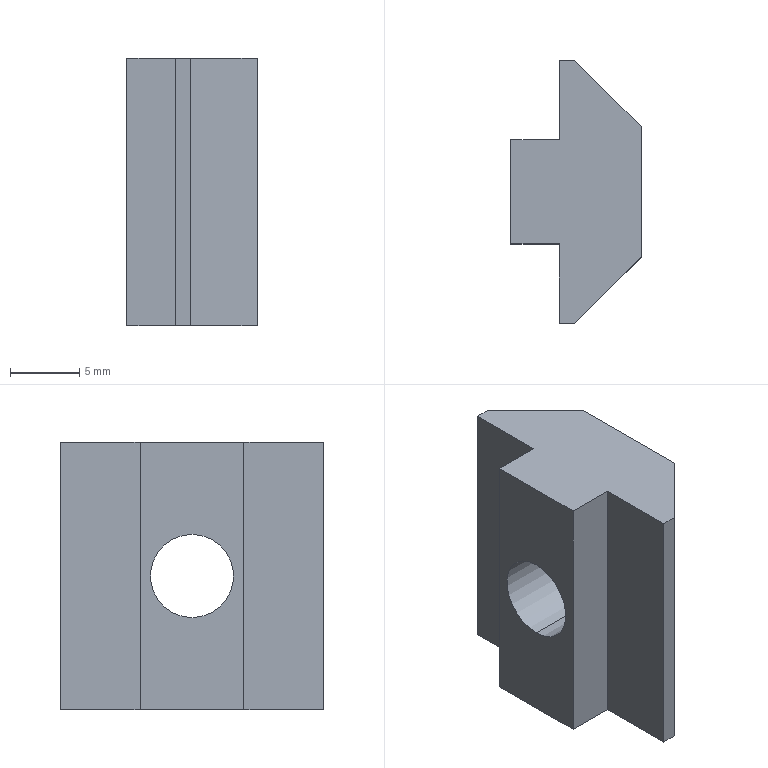Component | SolidWorks | SquareNutBlock-MC6-8-30-1 | 1 solid | 14 faces | box 9.4 x 19 x 19.3 mm | volume 1960 mm3 | plane 12 | cylinder 2 | commonest cylinder face diameters 6 x2 | material Purchased Part
build123d program:
from build123d import *

# Parameters (mm, degrees)
BOSS_EXTRUDE1_DEPTH = 9.65
M6_TAPPED_HOLE1_D   = 6


with BuildPart() as part:
    # Sketch1 → Boss-Extrude1 (new, symmetric)
    with BuildSketch(Plane.XY):
        Polygon((0, -3.75), (0, 3.75), (3.5, 3.75), (3.5, 9.5), (4.6, 9.5), (9.4, 4.7), (9.4, -4.7), (4.6, -9.5), (3.5, -9.5), (3.5, -3.75), align=None)
    extrude(amount=BOSS_EXTRUDE1_DEPTH, both=True)

    # M6 Tapped Hole1 (through all)
    with Locations(Plane(origin=(9.4, 0, 0), x_dir=(0, 0, -1), z_dir=(1, 0, 0))):
        with Locations((0, 0)):
            Hole(M6_TAPPED_HOLE1_D / 2)


solid = part.part

# Placed as in the assembly
solid = solid.moved(Location((11.4, -250, 10), (0, 0, 0)))
STEP:
#1=CARTESIAN_POINT('',(0.4488,-9.843,0.5118));
#2=VERTEX_POINT('',#1);
#3=CARTESIAN_POINT('',(0.4488,-9.843,0.2756));
#4=VERTEX_POINT('',#3);
#5=CARTESIAN_POINT('',(0.4488,-9.843,0.3937));
#6=DIRECTION('',(1.,0.,0.));
#7=DIRECTION('',(0.,0.,-1.));
#8=AXIS2_PLACEMENT_3D('',#5,#6,#7);
#9=CIRCLE('',#8,0.1181);
#10=EDGE_CURVE('',#2,#4,#9,.T.);
#11=ORIENTED_EDGE('',*,*,#10,.F.);
#12=CARTESIAN_POINT('',(0.8189,-9.843,0.5118));
#13=VERTEX_POINT('',#12);
#14=CARTESIAN_POINT('',(0.8189,-9.843,0.5118));
#15=DIRECTION('',(1.,0.,0.));
#16=VECTOR('',#15,39.37);
#17=LINE('',#14,#16);
#18=EDGE_CURVE('',#2,#13,#17,.T.);
#19=ORIENTED_EDGE('',*,*,#18,.T.);
#20=CARTESIAN_POINT('',(0.8189,-9.843,0.2756));
#21=VERTEX_POINT('',#20);
#22=CARTESIAN_POINT('',(0.8189,-9.843,0.3937));
#23=DIRECTION('',(1.,0.,0.));
#24=DIRECTION('',(0.,0.,-1.));
#25=AXIS2_PLACEMENT_3D('',#22,#23,#24);
#26=CIRCLE('',#25,0.1181);
#27=EDGE_CURVE('',#13,#21,#26,.T.);
#28=ORIENTED_EDGE('',*,*,#27,.T.);
#29=CARTESIAN_POINT('',(0.8189,-9.843,0.2756));
#30=DIRECTION('',(1.,0.,0.));
#31=VECTOR('',#30,39.37);
#32=LINE('',#29,#31);
#33=EDGE_CURVE('',#4,#21,#32,.T.);
#34=ORIENTED_EDGE('',*,*,#33,.F.);
#35=EDGE_LOOP('',(#11,#19,#28,#34));
#36=FACE_OUTER_BOUND('',#35,.T.);
#37=CARTESIAN_POINT('',(0.8189,-9.843,0.3937));
#38=DIRECTION('',(1.,0.,0.));
#39=DIRECTION('',(0.,0.,-1.));
#40=AXIS2_PLACEMENT_3D('',#37,#38,#39);
#41=CYLINDRICAL_SURFACE('',#40,0.1181);
#42=ADVANCED_FACE('',(#36),#41,.F.);
#43=CARTESIAN_POINT('',(0.4488,-9.99,0.01378));
#44=VERTEX_POINT('',#43);
#45=CARTESIAN_POINT('',(0.5866,-9.99,0.01378));
#46=VERTEX_POINT('',#45);
#47=CARTESIAN_POINT('',(0.5866,-9.99,0.01378));
#48=DIRECTION('',(1.,0.,0.));
#49=VECTOR('',#48,39.37);
#50=LINE('',#47,#49);
#51=EDGE_CURVE('',#44,#46,#50,.T.);
#52=ORIENTED_EDGE('',*,*,#51,.T.);
#53=CARTESIAN_POINT('',(0.5866,-9.99,0.7736));
#54=VERTEX_POINT('',#53);
#55=CARTESIAN_POINT('',(0.5866,-9.99,0.7736));
#56=DIRECTION('',(0.,0.,-1.));
#57=VECTOR('',#56,39.37);
#58=LINE('',#55,#57);
#59=EDGE_CURVE('',#54,#46,#58,.T.);
#60=ORIENTED_EDGE('',*,*,#59,.F.);
#61=CARTESIAN_POINT('',(0.4488,-9.99,0.7736));
#62=VERTEX_POINT('',#61);
#63=CARTESIAN_POINT('',(0.5866,-9.99,0.7736));
#64=DIRECTION('',(1.,0.,0.));
#65=VECTOR('',#64,39.37);
#66=LINE('',#63,#65);
#67=EDGE_CURVE('',#62,#54,#66,.T.);
#68=ORIENTED_EDGE('',*,*,#67,.F.);
#69=CARTESIAN_POINT('',(0.4488,-9.99,0.7736));
#70=DIRECTION('',(0.,0.,-1.));
#71=VECTOR('',#70,39.37);
#72=LINE('',#69,#71);
#73=EDGE_CURVE('',#62,#44,#72,.T.);
#74=ORIENTED_EDGE('',*,*,#73,.T.);
#75=EDGE_LOOP('',(#52,#60,#68,#74));
#76=FACE_OUTER_BOUND('',#75,.T.);
#77=CARTESIAN_POINT('',(0.5866,-9.99,0.7736));
#78=DIRECTION('',(0.,1.,0.));
#79=DIRECTION('',(0.,0.,1.));
#80=AXIS2_PLACEMENT_3D('',#77,#78,#79);
#81=PLANE('',#80);
#82=ADVANCED_FACE('',(#76),#81,.F.);
#83=CARTESIAN_POINT('',(0.5866,-10.217,0.01378));
#84=VERTEX_POINT('',#83);
#85=CARTESIAN_POINT('',(0.5866,-10.217,0.01378));
#86=DIRECTION('',(0.,-1.,0.));
#87=VECTOR('',#86,39.37);
#88=LINE('',#85,#87);
#89=EDGE_CURVE('',#46,#84,#88,.T.);
#90=ORIENTED_EDGE('',*,*,#89,.T.);
#91=CARTESIAN_POINT('',(0.5866,-10.217,0.7736));
#92=VERTEX_POINT('',#91);
#93=CARTESIAN_POINT('',(0.5866,-10.217,0.7736));
#94=DIRECTION('',(0.,0.,-1.));
#95=VECTOR('',#94,39.37);
#96=LINE('',#93,#95);
#97=EDGE_CURVE('',#92,#84,#96,.T.);
#98=ORIENTED_EDGE('',*,*,#97,.F.);
#99=CARTESIAN_POINT('',(0.5866,-10.217,0.7736));
#100=DIRECTION('',(0.,-1.,0.));
#101=VECTOR('',#100,39.37);
#102=LINE('',#99,#101);
#103=EDGE_CURVE('',#54,#92,#102,.T.);
#104=ORIENTED_EDGE('',*,*,#103,.F.);
#105=ORIENTED_EDGE('',*,*,#59,.T.);
#106=EDGE_LOOP('',(#90,#98,#104,#105));
#107=FACE_OUTER_BOUND('',#106,.T.);
#108=CARTESIAN_POINT('',(0.5866,-10.217,0.7736));
#109=DIRECTION('',(1.,0.,0.));
#110=DIRECTION('',(-0.,1.,0.));
#111=AXIS2_PLACEMENT_3D('',#108,#109,#110);
#112=PLANE('',#111);
#113=ADVANCED_FACE('',(#107),#112,.F.);
#114=CARTESIAN_POINT('',(0.6299,-10.217,0.01378));
#115=VERTEX_POINT('',#114);
#116=CARTESIAN_POINT('',(0.6299,-10.217,0.01378));
#117=DIRECTION('',(1.,0.,0.));
#118=VECTOR('',#117,39.37);
#119=LINE('',#116,#118);
#120=EDGE_CURVE('',#84,#115,#119,.T.);
#121=ORIENTED_EDGE('',*,*,#120,.T.);
#122=CARTESIAN_POINT('',(0.6299,-10.217,0.7736));
#123=VERTEX_POINT('',#122);
#124=CARTESIAN_POINT('',(0.6299,-10.217,0.7736));
#125=DIRECTION('',(0.,0.,-1.));
#126=VECTOR('',#125,39.37);
#127=LINE('',#124,#126);
#128=EDGE_CURVE('',#123,#115,#127,.T.);
#129=ORIENTED_EDGE('',*,*,#128,.F.);
#130=CARTESIAN_POINT('',(0.6299,-10.217,0.7736));
#131=DIRECTION('',(1.,0.,0.));
#132=VECTOR('',#131,39.37);
#133=LINE('',#130,#132);
#134=EDGE_CURVE('',#92,#123,#133,.T.);
#135=ORIENTED_EDGE('',*,*,#134,.F.);
#136=ORIENTED_EDGE('',*,*,#97,.T.);
#137=EDGE_LOOP('',(#121,#129,#135,#136));
#138=FACE_OUTER_BOUND('',#137,.T.);
#139=CARTESIAN_POINT('',(0.6299,-10.217,0.7736));
#140=DIRECTION('',(0.,1.,0.));
#141=DIRECTION('',(0.,0.,1.));
#142=AXIS2_PLACEMENT_3D('',#139,#140,#141);
#143=PLANE('',#142);
#144=ADVANCED_FACE('',(#138),#143,.F.);
#145=CARTESIAN_POINT('',(0.8189,-10.028,0.01378));
#146=VERTEX_POINT('',#145);
#147=CARTESIAN_POINT('',(0.8189,-10.028,0.01378));
#148=DIRECTION('',(0.7071,0.7071,0.));
#149=VECTOR('',#148,39.37);
#150=LINE('',#147,#149);
#151=EDGE_CURVE('',#115,#146,#150,.T.);
#152=ORIENTED_EDGE('',*,*,#151,.T.);
#153=CARTESIAN_POINT('',(0.8189,-10.028,0.7736));
#154=VERTEX_POINT('',#153);
#155=CARTESIAN_POINT('',(0.8189,-10.028,0.7736));
#156=DIRECTION('',(0.,0.,-1.));
#157=VECTOR('',#156,39.37);
#158=LINE('',#155,#157);
#159=EDGE_CURVE('',#154,#146,#158,.T.);
#160=ORIENTED_EDGE('',*,*,#159,.F.);
#161=CARTESIAN_POINT('',(0.8189,-10.028,0.7736));
#162=DIRECTION('',(0.7071,0.7071,0.));
#163=VECTOR('',#162,39.37);
#164=LINE('',#161,#163);
#165=EDGE_CURVE('',#123,#154,#164,.T.);
#166=ORIENTED_EDGE('',*,*,#165,.F.);
#167=ORIENTED_EDGE('',*,*,#128,.T.);
#168=EDGE_LOOP('',(#152,#160,#166,#167));
#169=FACE_OUTER_BOUND('',#168,.T.);
#170=CARTESIAN_POINT('',(0.8189,-10.028,0.7736));
#171=DIRECTION('',(-0.7071,0.7071,0.));
#172=DIRECTION('',(-0.7071,-0.7071,0.));
#173=AXIS2_PLACEMENT_3D('',#170,#171,#172);
#174=PLANE('',#173);
#175=ADVANCED_FACE('',(#169),#174,.F.);
#176=CARTESIAN_POINT('',(0.8189,-9.843,0.3937));
#177=DIRECTION('',(1.,0.,0.));
#178=DIRECTION('',(0.,0.,-1.));
#179=AXIS2_PLACEMENT_3D('',#176,#177,#178);
#180=CIRCLE('',#179,0.1181);
#181=EDGE_CURVE('',#21,#13,#180,.T.);
#182=ORIENTED_EDGE('',*,*,#181,.F.);
#183=ORIENTED_EDGE('',*,*,#27,.F.);
#184=EDGE_LOOP('',(#182,#183));
#185=FACE_BOUND('',#184,.T.);
#186=CARTESIAN_POINT('',(0.8189,-9.657,0.01378));
#187=VERTEX_POINT('',#186);
#188=CARTESIAN_POINT('',(0.8189,-9.657,0.01378));
#189=DIRECTION('',(0.,1.,0.));
#190=VECTOR('',#189,39.37);
#191=LINE('',#188,#190);
#192=EDGE_CURVE('',#146,#187,#191,.T.);
#193=ORIENTED_EDGE('',*,*,#192,.T.);
#194=CARTESIAN_POINT('',(0.8189,-9.657,0.7736));
#195=VERTEX_POINT('',#194);
#196=CARTESIAN_POINT('',(0.8189,-9.657,0.7736));
#197=DIRECTION('',(0.,0.,-1.));
#198=VECTOR('',#197,39.37);
#199=LINE('',#196,#198);
#200=EDGE_CURVE('',#195,#187,#199,.T.);
#201=ORIENTED_EDGE('',*,*,#200,.F.);
#202=CARTESIAN_POINT('',(0.8189,-9.657,0.7736));
#203=DIRECTION('',(0.,1.,0.));
#204=VECTOR('',#203,39.37);
#205=LINE('',#202,#204);
#206=EDGE_CURVE('',#154,#195,#205,.T.);
#207=ORIENTED_EDGE('',*,*,#206,.F.);
#208=ORIENTED_EDGE('',*,*,#159,.T.);
#209=EDGE_LOOP('',(#193,#201,#207,#208));
#210=FACE_OUTER_BOUND('',#209,.T.);
#211=CARTESIAN_POINT('',(0.8189,-9.657,0.7736));
#212=DIRECTION('',(-1.,0.,0.));
#213=DIRECTION('',(0.,0.,1.));
#214=AXIS2_PLACEMENT_3D('',#211,#212,#213);
#215=PLANE('',#214);
#216=ADVANCED_FACE('',(#185,#210),#215,.F.);
#217=CARTESIAN_POINT('',(0.6299,-9.469,0.01378));
#218=VERTEX_POINT('',#217);
#219=CARTESIAN_POINT('',(0.6299,-9.469,0.01378));
#220=DIRECTION('',(-0.7071,0.7071,0.));
#221=VECTOR('',#220,39.37);
#222=LINE('',#219,#221);
#223=EDGE_CURVE('',#187,#218,#222,.T.);
#224=ORIENTED_EDGE('',*,*,#223,.T.);
#225=CARTESIAN_POINT('',(0.6299,-9.469,0.7736));
#226=VERTEX_POINT('',#225);
#227=CARTESIAN_POINT('',(0.6299,-9.469,0.7736));
#228=DIRECTION('',(0.,0.,-1.));
#229=VECTOR('',#228,39.37);
#230=LINE('',#227,#229);
#231=EDGE_CURVE('',#226,#218,#230,.T.);
#232=ORIENTED_EDGE('',*,*,#231,.F.);
#233=CARTESIAN_POINT('',(0.6299,-9.469,0.7736));
#234=DIRECTION('',(-0.7071,0.7071,0.));
#235=VECTOR('',#234,39.37);
#236=LINE('',#233,#235);
#237=EDGE_CURVE('',#195,#226,#236,.T.);
#238=ORIENTED_EDGE('',*,*,#237,.F.);
#239=ORIENTED_EDGE('',*,*,#200,.T.);
#240=EDGE_LOOP('',(#224,#232,#238,#239));
#241=FACE_OUTER_BOUND('',#240,.T.);
#242=CARTESIAN_POINT('',(0.6299,-9.469,0.7736));
#243=DIRECTION('',(-0.7071,-0.7071,0.));
#244=DIRECTION('',(0.7071,-0.7071,0.));
#245=AXIS2_PLACEMENT_3D('',#242,#243,#244);
#246=PLANE('',#245);
#247=ADVANCED_FACE('',(#241),#246,.F.);
#248=CARTESIAN_POINT('',(0.5866,-9.469,0.01378));
#249=VERTEX_POINT('',#248);
#250=CARTESIAN_POINT('',(0.5866,-9.469,0.01378));
#251=DIRECTION('',(-1.,0.,0.));
#252=VECTOR('',#251,39.37);
#253=LINE('',#250,#252);
#254=EDGE_CURVE('',#218,#249,#253,.T.);
#255=ORIENTED_EDGE('',*,*,#254,.T.);
#256=CARTESIAN_POINT('',(0.5866,-9.469,0.7736));
#257=VERTEX_POINT('',#256);
#258=CARTESIAN_POINT('',(0.5866,-9.469,0.7736));
#259=DIRECTION('',(0.,0.,-1.));
#260=VECTOR('',#259,39.37);
#261=LINE('',#258,#260);
#262=EDGE_CURVE('',#257,#249,#261,.T.);
#263=ORIENTED_EDGE('',*,*,#262,.F.);
#264=CARTESIAN_POINT('',(0.5866,-9.469,0.7736));
#265=DIRECTION('',(-1.,0.,0.));
#266=VECTOR('',#265,39.37);
#267=LINE('',#264,#266);
#268=EDGE_CURVE('',#226,#257,#267,.T.);
#269=ORIENTED_EDGE('',*,*,#268,.F.);
#270=ORIENTED_EDGE('',*,*,#231,.T.);
#271=EDGE_LOOP('',(#255,#263,#269,#270));
#272=FACE_OUTER_BOUND('',#271,.T.);
#273=CARTESIAN_POINT('',(0.5866,-9.469,0.7736));
#274=DIRECTION('',(0.,-1.,0.));
#275=DIRECTION('',(0.,0.,-1.));
#276=AXIS2_PLACEMENT_3D('',#273,#274,#275);
#277=PLANE('',#276);
#278=ADVANCED_FACE('',(#272),#277,.F.);
#279=CARTESIAN_POINT('',(0.5866,-9.695,0.01378));
#280=VERTEX_POINT('',#279);
#281=CARTESIAN_POINT('',(0.5866,-9.695,0.01378));
#282=DIRECTION('',(-0.,-1.,0.));
#283=VECTOR('',#282,39.37);
#284=LINE('',#281,#283);
#285=EDGE_CURVE('',#249,#280,#284,.T.);
#286=ORIENTED_EDGE('',*,*,#285,.T.);
#287=CARTESIAN_POINT('',(0.5866,-9.695,0.7736));
#288=VERTEX_POINT('',#287);
#289=CARTESIAN_POINT('',(0.5866,-9.695,0.7736));
#290=DIRECTION('',(0.,0.,-1.));
#291=VECTOR('',#290,39.37);
#292=LINE('',#289,#291);
#293=EDGE_CURVE('',#288,#280,#292,.T.);
#294=ORIENTED_EDGE('',*,*,#293,.F.);
#295=CARTESIAN_POINT('',(0.5866,-9.695,0.7736));
#296=DIRECTION('',(-0.,-1.,0.));
#297=VECTOR('',#296,39.37);
#298=LINE('',#295,#297);
#299=EDGE_CURVE('',#257,#288,#298,.T.);
#300=ORIENTED_EDGE('',*,*,#299,.F.);
#301=ORIENTED_EDGE('',*,*,#262,.T.);
#302=EDGE_LOOP('',(#286,#294,#300,#301));
#303=FACE_OUTER_BOUND('',#302,.T.);
#304=CARTESIAN_POINT('',(0.5866,-9.695,0.7736));
#305=DIRECTION('',(1.,-0.,0.));
#306=DIRECTION('',(0.,1.,0.));
#307=AXIS2_PLACEMENT_3D('',#304,#305,#306);
#308=PLANE('',#307);
#309=ADVANCED_FACE('',(#303),#308,.F.);
#310=CARTESIAN_POINT('',(0.4488,-9.695,0.01378));
#311=VERTEX_POINT('',#310);
#312=CARTESIAN_POINT('',(0.4488,-9.695,0.01378));
#313=DIRECTION('',(-1.,0.,0.));
#314=VECTOR('',#313,39.37);
#315=LINE('',#312,#314);
#316=EDGE_CURVE('',#280,#311,#315,.T.);
#317=ORIENTED_EDGE('',*,*,#316,.T.);
#318=CARTESIAN_POINT('',(0.4488,-9.695,0.7736));
#319=VERTEX_POINT('',#318);
#320=CARTESIAN_POINT('',(0.4488,-9.695,0.7736));
#321=DIRECTION('',(0.,0.,-1.));
#322=VECTOR('',#321,39.37);
#323=LINE('',#320,#322);
#324=EDGE_CURVE('',#319,#311,#323,.T.);
#325=ORIENTED_EDGE('',*,*,#324,.F.);
#326=CARTESIAN_POINT('',(0.4488,-9.695,0.7736));
#327=DIRECTION('',(-1.,0.,0.));
#328=VECTOR('',#327,39.37);
#329=LINE('',#326,#328);
#330=EDGE_CURVE('',#288,#319,#329,.T.);
#331=ORIENTED_EDGE('',*,*,#330,.F.);
#332=ORIENTED_EDGE('',*,*,#293,.T.);
#333=EDGE_LOOP('',(#317,#325,#331,#332));
#334=FACE_OUTER_BOUND('',#333,.T.);
#335=CARTESIAN_POINT('',(0.4488,-9.695,0.7736));
#336=DIRECTION('',(0.,-1.,0.));
#337=DIRECTION('',(0.,0.,-1.));
#338=AXIS2_PLACEMENT_3D('',#335,#336,#337);
#339=PLANE('',#338);
#340=ADVANCED_FACE('',(#334),#339,.F.);
#341=CARTESIAN_POINT('',(0.4488,-9.843,0.3937));
#342=DIRECTION('',(1.,0.,0.));
#343=DIRECTION('',(0.,0.,-1.));
#344=AXIS2_PLACEMENT_3D('',#341,#342,#343);
#345=CIRCLE('',#344,0.1181);
#346=EDGE_CURVE('',#4,#2,#345,.T.);
#347=ORIENTED_EDGE('',*,*,#346,.T.);
#348=ORIENTED_EDGE('',*,*,#10,.T.);
#349=EDGE_LOOP('',(#347,#348));
#350=FACE_BOUND('',#349,.T.);
#351=CARTESIAN_POINT('',(0.4488,-9.99,0.01378));
#352=DIRECTION('',(0.,-1.,0.));
#353=VECTOR('',#352,39.37);
#354=LINE('',#351,#353);
#355=EDGE_CURVE('',#311,#44,#354,.T.);
#356=ORIENTED_EDGE('',*,*,#355,.T.);
#357=ORIENTED_EDGE('',*,*,#73,.F.);
#358=CARTESIAN_POINT('',(0.4488,-9.99,0.7736));
#359=DIRECTION('',(0.,-1.,0.));
#360=VECTOR('',#359,39.37);
#361=LINE('',#358,#360);
#362=EDGE_CURVE('',#319,#62,#361,.T.);
#363=ORIENTED_EDGE('',*,*,#362,.F.);
#364=ORIENTED_EDGE('',*,*,#324,.T.);
#365=EDGE_LOOP('',(#356,#357,#363,#364));
#366=FACE_OUTER_BOUND('',#365,.T.);
#367=CARTESIAN_POINT('',(0.4488,-9.99,0.7736));
#368=DIRECTION('',(1.,0.,0.));
#369=DIRECTION('',(0.,0.,-1.));
#370=AXIS2_PLACEMENT_3D('',#367,#368,#369);
#371=PLANE('',#370);
#372=ADVANCED_FACE('',(#350,#366),#371,.F.);
#373=ORIENTED_EDGE('',*,*,#67,.T.);
#374=ORIENTED_EDGE('',*,*,#103,.T.);
#375=ORIENTED_EDGE('',*,*,#134,.T.);
#376=ORIENTED_EDGE('',*,*,#165,.T.);
#377=ORIENTED_EDGE('',*,*,#206,.T.);
#378=ORIENTED_EDGE('',*,*,#237,.T.);
#379=ORIENTED_EDGE('',*,*,#268,.T.);
#380=ORIENTED_EDGE('',*,*,#299,.T.);
#381=ORIENTED_EDGE('',*,*,#330,.T.);
#382=ORIENTED_EDGE('',*,*,#362,.T.);
#383=EDGE_LOOP('',(#373,#374,#375,#376,#377,#378,#379,#380,#381,#382));
#384=FACE_OUTER_BOUND('',#383,.T.);
#385=CARTESIAN_POINT('',(0.4488,-9.843,0.7736));
#386=DIRECTION('',(0.,0.,-1.));
#387=DIRECTION('',(-1.,0.,0.));
#388=AXIS2_PLACEMENT_3D('',#385,#386,#387);
#389=PLANE('',#388);
#390=ADVANCED_FACE('',(#384),#389,.F.);
#391=ORIENTED_EDGE('',*,*,#51,.F.);
#392=ORIENTED_EDGE('',*,*,#355,.F.);
#393=ORIENTED_EDGE('',*,*,#316,.F.);
#394=ORIENTED_EDGE('',*,*,#285,.F.);
#395=ORIENTED_EDGE('',*,*,#254,.F.);
#396=ORIENTED_EDGE('',*,*,#223,.F.);
#397=ORIENTED_EDGE('',*,*,#192,.F.);
#398=ORIENTED_EDGE('',*,*,#151,.F.);
#399=ORIENTED_EDGE('',*,*,#120,.F.);
#400=ORIENTED_EDGE('',*,*,#89,.F.);
#401=EDGE_LOOP('',(#391,#392,#393,#394,#395,#396,#397,#398,#399,#400));
#402=FACE_OUTER_BOUND('',#401,.T.);
#403=CARTESIAN_POINT('',(0.4488,-9.843,0.01378));
#404=DIRECTION('',(0.,0.,-1.));
#405=DIRECTION('',(-1.,0.,0.));
#406=AXIS2_PLACEMENT_3D('',#403,#404,#405);
#407=PLANE('',#406);
#408=ADVANCED_FACE('',(#402),#407,.T.);
#409=ORIENTED_EDGE('',*,*,#18,.F.);
#410=ORIENTED_EDGE('',*,*,#346,.F.);
#411=ORIENTED_EDGE('',*,*,#33,.T.);
#412=ORIENTED_EDGE('',*,*,#181,.T.);
#413=EDGE_LOOP('',(#409,#410,#411,#412));
#414=FACE_OUTER_BOUND('',#413,.T.);
#415=CARTESIAN_POINT('',(0.8189,-9.843,0.3937));
#416=DIRECTION('',(1.,0.,0.));
#417=DIRECTION('',(0.,0.,-1.));
#418=AXIS2_PLACEMENT_3D('',#415,#416,#417);
#419=CYLINDRICAL_SURFACE('',#418,0.1181);
#420=ADVANCED_FACE('',(#414),#419,.F.);
#421=CLOSED_SHELL('',(#42,#82,#113,#144,#175,#216,#247,#278,#309,#340,#372,#390,#408,#420));
#422=MANIFOLD_SOLID_BREP('',#421);
#423=CARTESIAN_POINT('',(0.,0.,0.));
#424=DIRECTION('',(0.,0.,1.));
#425=DIRECTION('',(1.,0.,0.));
#426=AXIS2_PLACEMENT_3D('',#423,#424,#425);
#427=(LENGTH_UNIT()NAMED_UNIT(*)SI_UNIT($,.METRE.));
#428=LENGTH_MEASURE_WITH_UNIT(LENGTH_MEASURE(0.0254),#427);
#429=DIMENSIONAL_EXPONENTS(1.,0.,0.,0.,0.,0.,0.);
#430=(CONVERSION_BASED_UNIT('',#428)LENGTH_UNIT()NAMED_UNIT(#429));
#431=UNCERTAINTY_MEASURE_WITH_UNIT(LENGTH_MEASURE(0.00001),#430,'','');
#432=(NAMED_UNIT(*)PLANE_ANGLE_UNIT()SI_UNIT($,.RADIAN.));
#433=(NAMED_UNIT(*)SI_UNIT($,.STERADIAN.)SOLID_ANGLE_UNIT());
#434=(GEOMETRIC_REPRESENTATION_CONTEXT(3)GLOBAL_UNCERTAINTY_ASSIGNED_CONTEXT((#431))GLOBAL_UNIT_ASSIGNED_CONTEXT((#430,#432,#433))REPRESENTATION_CONTEXT('',''));
#435=ADVANCED_BREP_SHAPE_REPRESENTATION('',(#422,#426),#434);
#436=COLOUR_RGB('',0.7922,0.8196,0.9333);
#437=FILL_AREA_STYLE_COLOUR('',#436);
#438=FILL_AREA_STYLE('',(#437));
#439=SURFACE_STYLE_FILL_AREA(#438);
#440=SURFACE_SIDE_STYLE('',(#439));
#441=SURFACE_STYLE_USAGE(.BOTH.,#440);
#442=PRESENTATION_STYLE_ASSIGNMENT((#441));
#443=STYLED_ITEM('',(#442),#422);
#444=PRESENTATION_LAYER_ASSIGNMENT('','',(#443));
#445=(LENGTH_UNIT()NAMED_UNIT(*)SI_UNIT($,.METRE.));
#446=LENGTH_MEASURE_WITH_UNIT(LENGTH_MEASURE(0.0254),#445);
#447=DIMENSIONAL_EXPONENTS(1.,0.,0.,0.,0.,0.,0.);
#448=(CONVERSION_BASED_UNIT('',#446)LENGTH_UNIT()NAMED_UNIT(#447));
#449=UNCERTAINTY_MEASURE_WITH_UNIT(LENGTH_MEASURE(0.00001),#448,'','');
#450=(NAMED_UNIT(*)PLANE_ANGLE_UNIT()SI_UNIT($,.RADIAN.));
#451=(NAMED_UNIT(*)SI_UNIT($,.STERADIAN.)SOLID_ANGLE_UNIT());
#452=(GEOMETRIC_REPRESENTATION_CONTEXT(3)GLOBAL_UNCERTAINTY_ASSIGNED_CONTEXT((#449))GLOBAL_UNIT_ASSIGNED_CONTEXT((#448,#450,#451))REPRESENTATION_CONTEXT('',''));
#453=MECHANICAL_DESIGN_GEOMETRIC_PRESENTATION_REPRESENTATION('',(#443),#452);